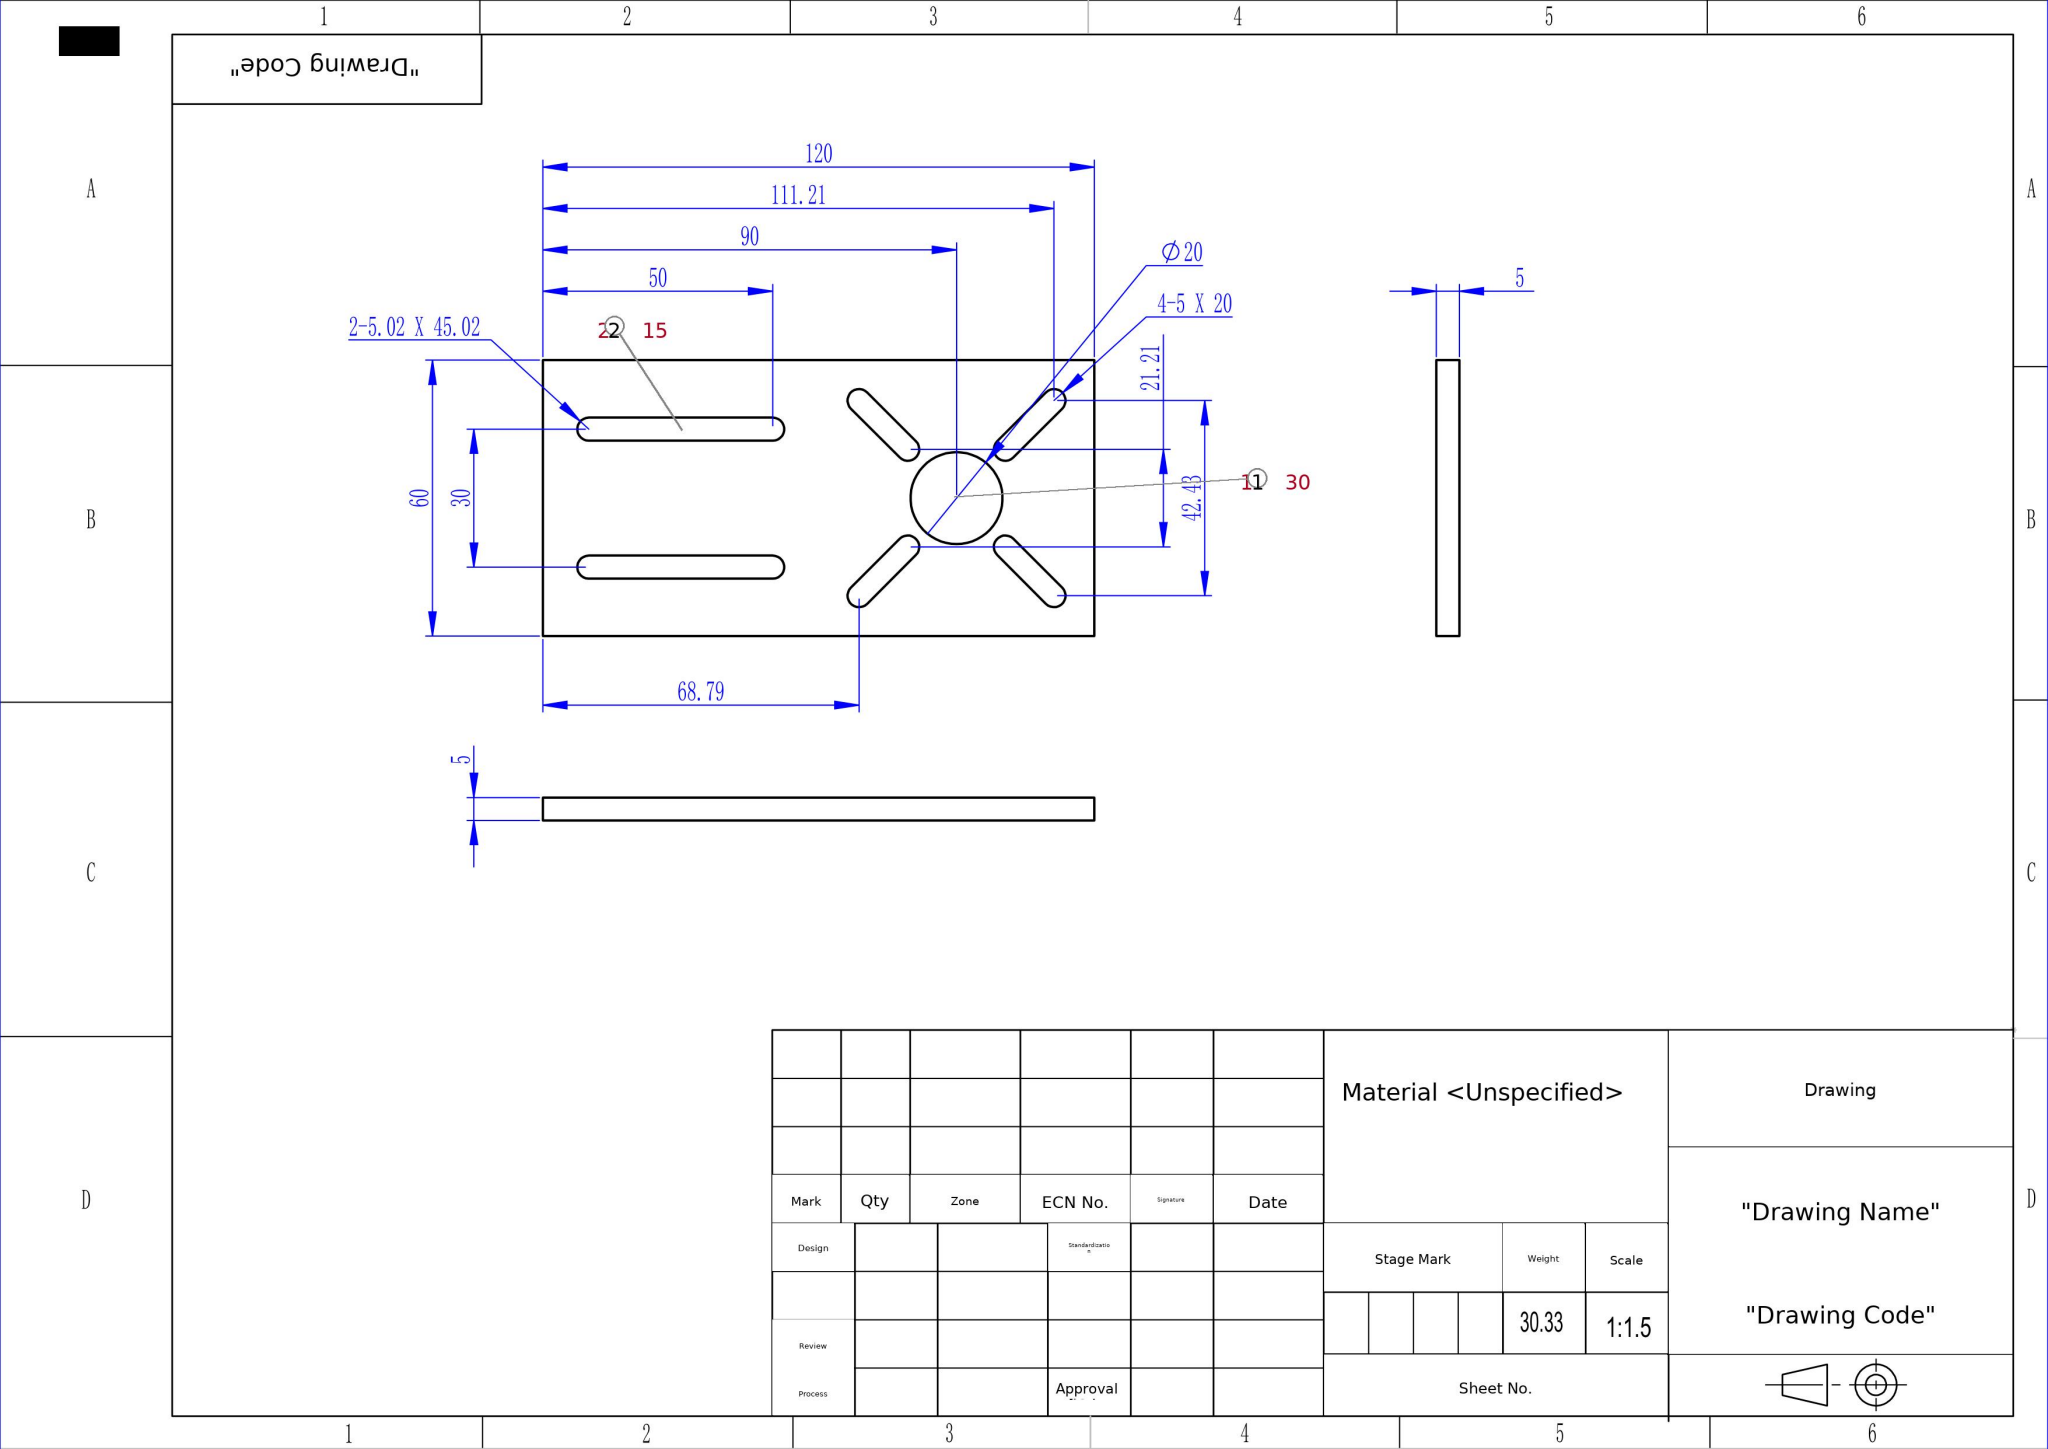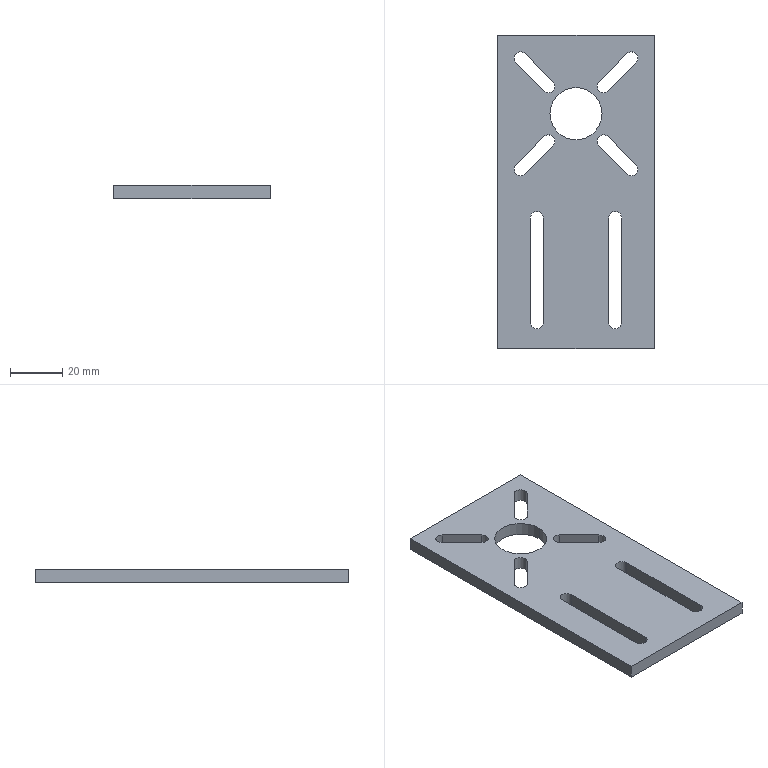Part | SolidWorks | mm | 1 solid | 36 faces | box 60 x 120 x 5 mm | volume 30331 mm3 | cylinder 18 | plane 18 | commonest cylinder face diameters 5 x12 5.02 x4 20 x2
build123d program:
from build123d import *

# Parameters (mm, degrees)
SKETCH1_W           = 30
SKETCH1_H           = 60
BOSS_EXTRUDE1_DEPTH = 5


with BuildPart() as part:
    # Sketch1 → Boss-Extrude1 (new body)
    # profile 1 of 10: a face of its own
    with BuildSketch(Plane.XY):
        with BuildLine():
            Line((0, 40), (0, 60))
            Line((0, 60), (-30, 60))
            Line((-30, 60), (-22.981, 52.981))
            ThreePointArc((-22.981, 52.981), (-21.213, 53.713), (-19.445, 52.981))
            Line((-19.445, 52.981), (-8.839, 42.374))
            ThreePointArc((-8.839, 42.374), (-8.107, 40.607), (-8.839, 38.839))
            Line((-8.839, 38.839), (-7.071, 37.071))
            ThreePointArc((-7.071, 37.071), (-3.827, 39.239), (0, 40))
        make_face()
    # profile 2 of 10: a face of its own
    with BuildSketch(Plane.XY):
        with BuildLine():
            Line((-30, 60), (-30, 30))
            Line((-30, 30), (-10, 30))
            ThreePointArc((-10, 30), (-9.239, 33.827), (-7.071, 37.071))
            Line((-7.071, 37.071), (-8.839, 38.839))
            ThreePointArc((-8.839, 38.839), (-10.607, 38.107), (-12.374, 38.839))
            Line((-12.374, 38.839), (-22.981, 49.445))
            ThreePointArc((-22.981, 49.445), (-23.713, 51.213), (-22.981, 52.981))
            Line((-22.981, 52.981), (-30, 60))
        make_face()
    # profile 3 of 10: a face of its own
    with BuildSketch(Plane.XY):
        with BuildLine():
            Line((22.981, 52.981), (30, 60))
            Line((30, 60), (0, 60))
            Line((0, 60), (0, 40))
            ThreePointArc((0, 40), (3.827, 39.239), (7.071, 37.071))
            Line((7.071, 37.071), (8.839, 38.839))
            ThreePointArc((8.839, 38.839), (8.107, 40.607), (8.839, 42.374))
            Line((8.839, 42.374), (19.445, 52.981))
            ThreePointArc((19.445, 52.981), (21.213, 53.713), (22.981, 52.981))
        make_face()
    # profile 4 of 10: a face of its own
    with BuildSketch(Plane.XY):
        with BuildLine():
            Line((10, 30), (30, 30))
            Line((30, 30), (30, 60))
            Line((30, 60), (22.981, 52.981))
            ThreePointArc((22.981, 52.981), (23.713, 51.213), (22.981, 49.445))
            Line((22.981, 49.445), (12.374, 38.839))
            ThreePointArc((12.374, 38.839), (10.607, 38.107), (8.839, 38.839))
            Line((8.839, 38.839), (7.071, 37.071))
            ThreePointArc((7.071, 37.071), (9.239, 33.827), (10, 30))
        make_face()
    # profile 5 of 10: a face of its own
    with BuildSketch(Plane.XY):
        with BuildLine():
            Line((-30, 30), (-30, 0))
            Line((-30, 0), (-22.981, 7.019))
            ThreePointArc((-22.981, 7.019), (-23.713, 8.787), (-22.981, 10.555))
            Line((-22.981, 10.555), (-12.374, 21.161))
            ThreePointArc((-12.374, 21.161), (-10.607, 21.893), (-8.839, 21.161))
            Line((-8.839, 21.161), (-7.071, 22.929))
            ThreePointArc((-7.071, 22.929), (-9.239, 26.173), (-10, 30))
            Line((-10, 30), (-30, 30))
        make_face()
    # profile 6 of 10: a face of its own
    with BuildSketch(Plane.XY):
        with BuildLine():
            Line((-30, 0), (0, 0))
            Line((0, 0), (0, 20))
            ThreePointArc((0, 20), (-3.827, 20.761), (-7.071, 22.929))
            Line((-7.071, 22.929), (-8.839, 21.161))
            ThreePointArc((-8.839, 21.161), (-8.107, 19.393), (-8.839, 17.626))
            Line((-8.839, 17.626), (-19.445, 7.019))
            ThreePointArc((-19.445, 7.019), (-21.213, 6.287), (-22.981, 7.019))
            Line((-22.981, 7.019), (-30, 0))
        make_face()
    # profile 7 of 10: a face of its own
    with BuildSketch(Plane.XY):
        with BuildLine():
            Line((0, 0), (30, 0))
            Line((30, 0), (22.981, 7.019))
            ThreePointArc((22.981, 7.019), (21.213, 6.287), (19.445, 7.019))
            Line((19.445, 7.019), (8.839, 17.626))
            ThreePointArc((8.839, 17.626), (8.107, 19.393), (8.839, 21.161))
            Line((8.839, 21.161), (7.071, 22.929))
            ThreePointArc((7.071, 22.929), (3.827, 20.761), (0, 20))
            Line((0, 20), (0, 0))
        make_face()
    # profile 8 of 10: a face of its own
    with BuildSketch(Plane.XY):
        with BuildLine():
            Line((22.981, 7.019), (30, 0))
            Line((30, 0), (30, 30))
            Line((30, 30), (10, 30))
            ThreePointArc((10, 30), (9.239, 26.173), (7.071, 22.929))
            Line((7.071, 22.929), (8.839, 21.161))
            ThreePointArc((8.839, 21.161), (10.607, 21.893), (12.374, 21.161))
            Line((12.374, 21.161), (22.981, 10.555))
            ThreePointArc((22.981, 10.555), (23.713, 8.787), (22.981, 7.019))
        make_face()
    # profile 9 of 10: a face of its own
    with BuildSketch(Plane.XY):
        with Locations((15, -30)):
            Rectangle(SKETCH1_W, SKETCH1_H)
        with BuildLine():
            Line((12.49, -50), (12.49, -10))
            ThreePointArc((12.49, -10), (15, -7.49), (17.51, -10))
            Line((17.51, -10), (17.51, -50))
            ThreePointArc((17.51, -50), (15, -52.51), (12.49, -50))
        make_face(mode=Mode.SUBTRACT)
    # profile 10 of 10: a face of its own
    with BuildSketch(Plane.XY):
        with Locations((-15, -30)):
            Rectangle(SKETCH1_W, SKETCH1_H)
        with BuildLine():
            ThreePointArc((-17.51, -10), (-15, -7.49), (-12.49, -10))
            Line((-12.49, -10), (-12.49, -50))
            ThreePointArc((-12.49, -50), (-15, -52.51), (-17.51, -50))
            Line((-17.51, -50), (-17.51, -10))
        make_face(mode=Mode.SUBTRACT)
    extrude(amount=BOSS_EXTRUDE1_DEPTH)


solid = part.part